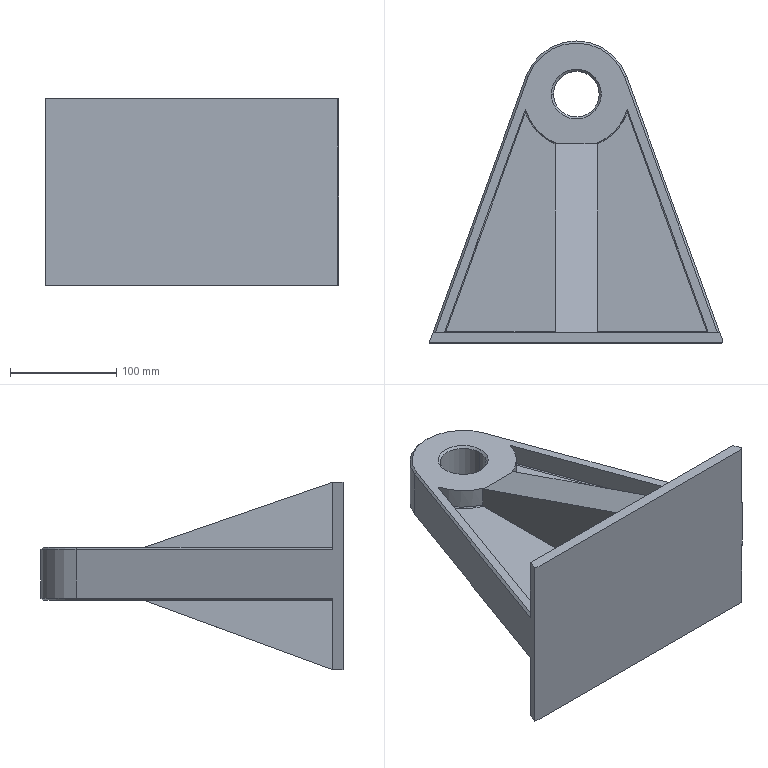Component | SolidWorks | SupportBase2-2 | 1 solid | 59 faces | volume 2355379 mm3 | plane 34 | cylinder 15 | cone 6 | torus 4 | commonest cylinder face diameters 2 x8 100 x5 43 x2 | material 45